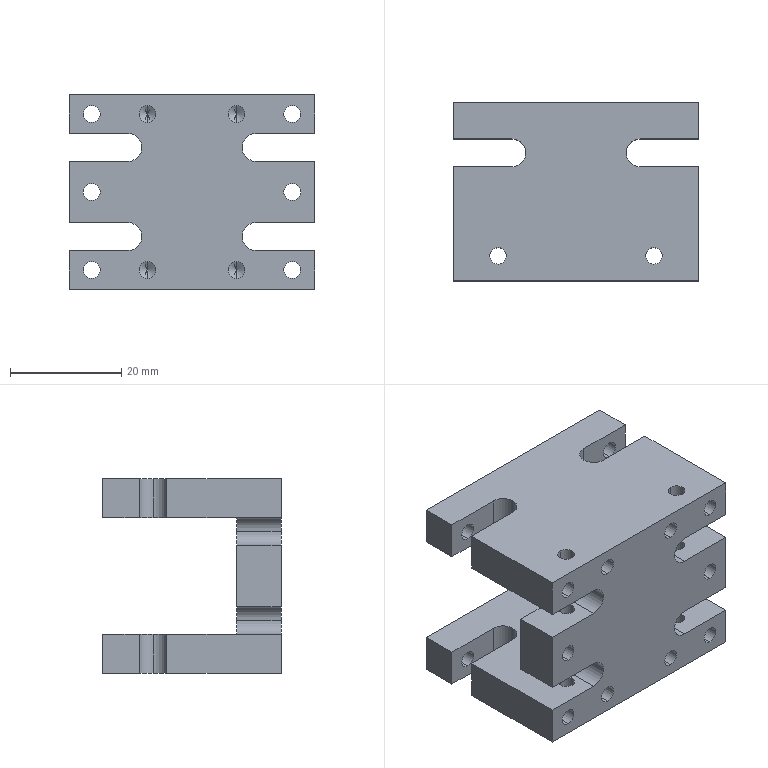Component | SolidWorks | BeamSlidingPair-1 | 1 solid | 94 faces | volume 21844 mm3 | cylinder 56 | plane 30 | cone 8 | commonest cylinder face diameters 3 x40 5 x16 | material 6061 Alloy